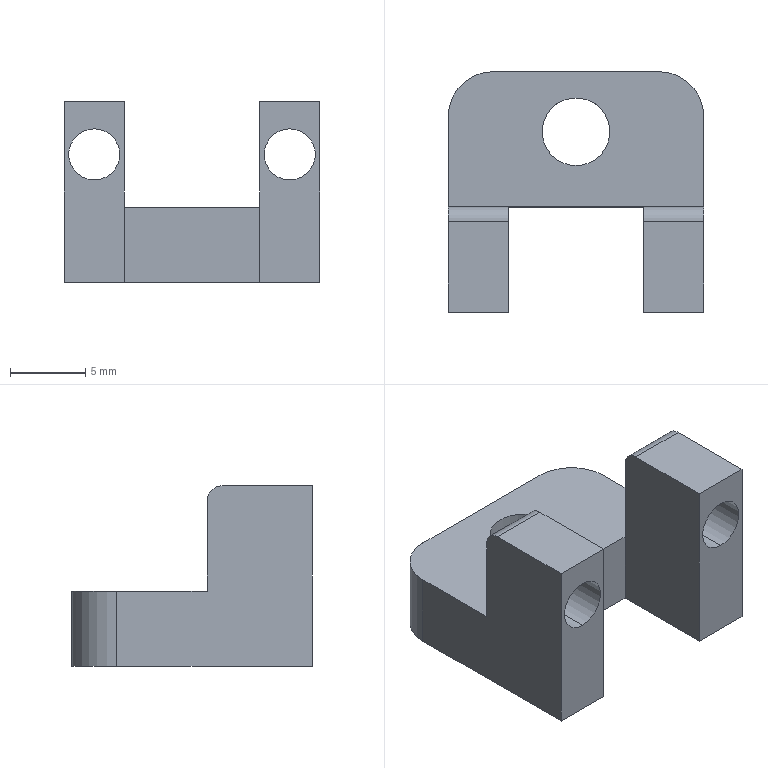Component | SolidWorks | MGL-PACK-01-00WeldedPlate1Assembly-1_MGL-PACK-01-03FixingBlock-1 | 1 solid | 24 faces | box 17 x 16 x 12 mm | volume 1209 mm3 | plane 14 | cylinder 10 | commonest cylinder face diameters 3.4 x4 4.5 x2 6 x2 2 x2
STEP:
#1=COLOUR_RGB('',0.7922,0.8196,0.9333);
#2=FILL_AREA_STYLE_COLOUR('',#1);
#3=FILL_AREA_STYLE('',(#2));
#4=SURFACE_STYLE_FILL_AREA(#3);
#5=SURFACE_SIDE_STYLE('',(#4));
#6=SURFACE_STYLE_USAGE(.BOTH.,#5);
#7=PRESENTATION_STYLE_ASSIGNMENT((#6));
#8=CARTESIAN_POINT('',(-3.585,1.831,0.2677));
#9=VERTEX_POINT('',#8);
#10=CARTESIAN_POINT('',(-3.585,1.831,0.4016));
#11=VERTEX_POINT('',#10);
#12=CARTESIAN_POINT('',(-3.585,1.831,0.3346));
#13=DIRECTION('',(-0.,1.,0.));
#14=DIRECTION('',(-1.,0.,0.));
#15=AXIS2_PLACEMENT_3D('',#12,#13,#14);
#16=CIRCLE('',#15,0.06693);
#17=EDGE_CURVE('',#9,#11,#16,.T.);
#18=ORIENTED_EDGE('',*,*,#17,.F.);
#19=CARTESIAN_POINT('',(-3.585,2.106,0.2677));
#20=VERTEX_POINT('',#19);
#21=CARTESIAN_POINT('',(-3.585,2.106,0.2677));
#22=DIRECTION('',(0.,1.,0.));
#23=VECTOR('',#22,39.37);
#24=LINE('',#21,#23);
#25=EDGE_CURVE('',#9,#20,#24,.T.);
#26=ORIENTED_EDGE('',*,*,#25,.T.);
#27=CARTESIAN_POINT('',(-3.585,2.106,0.4016));
#28=VERTEX_POINT('',#27);
#29=CARTESIAN_POINT('',(-3.585,2.106,0.3346));
#30=DIRECTION('',(0.,1.,0.));
#31=DIRECTION('',(0.,0.,1.));
#32=AXIS2_PLACEMENT_3D('',#29,#30,#31);
#33=CIRCLE('',#32,0.06693);
#34=EDGE_CURVE('',#20,#28,#33,.T.);
#35=ORIENTED_EDGE('',*,*,#34,.T.);
#36=CARTESIAN_POINT('',(-3.585,2.106,0.4016));
#37=DIRECTION('',(0.,1.,0.));
#38=VECTOR('',#37,39.37);
#39=LINE('',#36,#38);
#40=EDGE_CURVE('',#11,#28,#39,.T.);
#41=ORIENTED_EDGE('',*,*,#40,.F.);
#42=EDGE_LOOP('',(#18,#26,#35,#41));
#43=FACE_OUTER_BOUND('',#42,.T.);
#44=CARTESIAN_POINT('',(-3.585,2.106,0.3346));
#45=DIRECTION('',(0.,1.,0.));
#46=DIRECTION('',(0.,0.,1.));
#47=AXIS2_PLACEMENT_3D('',#44,#45,#46);
#48=CYLINDRICAL_SURFACE('',#47,0.06693);
#49=ADVANCED_FACE('',(#43),#48,.F.);
#50=CARTESIAN_POINT('',(-3.073,1.831,0.2677));
#51=VERTEX_POINT('',#50);
#52=CARTESIAN_POINT('',(-3.073,1.831,0.4016));
#53=VERTEX_POINT('',#52);
#54=CARTESIAN_POINT('',(-3.073,1.831,0.3346));
#55=DIRECTION('',(0.,1.,0.));
#56=DIRECTION('',(-1.,0.,0.));
#57=AXIS2_PLACEMENT_3D('',#54,#55,#56);
#58=CIRCLE('',#57,0.06693);
#59=EDGE_CURVE('',#51,#53,#58,.T.);
#60=ORIENTED_EDGE('',*,*,#59,.F.);
#61=CARTESIAN_POINT('',(-3.073,2.106,0.2677));
#62=VERTEX_POINT('',#61);
#63=CARTESIAN_POINT('',(-3.073,2.106,0.2677));
#64=DIRECTION('',(0.,1.,0.));
#65=VECTOR('',#64,39.37);
#66=LINE('',#63,#65);
#67=EDGE_CURVE('',#51,#62,#66,.T.);
#68=ORIENTED_EDGE('',*,*,#67,.T.);
#69=CARTESIAN_POINT('',(-3.073,2.106,0.4016));
#70=VERTEX_POINT('',#69);
#71=CARTESIAN_POINT('',(-3.073,2.106,0.3346));
#72=DIRECTION('',(0.,1.,0.));
#73=DIRECTION('',(0.,0.,1.));
#74=AXIS2_PLACEMENT_3D('',#71,#72,#73);
#75=CIRCLE('',#74,0.06693);
#76=EDGE_CURVE('',#62,#70,#75,.T.);
#77=ORIENTED_EDGE('',*,*,#76,.T.);
#78=CARTESIAN_POINT('',(-3.073,2.106,0.4016));
#79=DIRECTION('',(0.,1.,0.));
#80=VECTOR('',#79,39.37);
#81=LINE('',#78,#80);
#82=EDGE_CURVE('',#53,#70,#81,.T.);
#83=ORIENTED_EDGE('',*,*,#82,.F.);
#84=EDGE_LOOP('',(#60,#68,#77,#83));
#85=FACE_OUTER_BOUND('',#84,.T.);
#86=CARTESIAN_POINT('',(-3.073,2.106,0.3346));
#87=DIRECTION('',(0.,1.,0.));
#88=DIRECTION('',(0.,0.,1.));
#89=AXIS2_PLACEMENT_3D('',#86,#87,#88);
#90=CYLINDRICAL_SURFACE('',#89,0.06693);
#91=ADVANCED_FACE('',(#85),#90,.F.);
#92=CARTESIAN_POINT('',(-3.417,2.303,0.));
#93=VERTEX_POINT('',#92);
#94=CARTESIAN_POINT('',(-3.24,2.303,0.));
#95=VERTEX_POINT('',#94);
#96=CARTESIAN_POINT('',(-3.329,2.303,0.));
#97=DIRECTION('',(0.,0.,1.));
#98=DIRECTION('',(1.,0.,0.));
#99=AXIS2_PLACEMENT_3D('',#96,#97,#98);
#100=CIRCLE('',#99,0.08858);
#101=EDGE_CURVE('',#93,#95,#100,.T.);
#102=ORIENTED_EDGE('',*,*,#101,.F.);
#103=CARTESIAN_POINT('',(-3.417,2.303,0.1969));
#104=VERTEX_POINT('',#103);
#105=CARTESIAN_POINT('',(-3.417,2.303,0.1969));
#106=DIRECTION('',(0.,0.,1.));
#107=VECTOR('',#106,39.37);
#108=LINE('',#105,#107);
#109=EDGE_CURVE('',#93,#104,#108,.T.);
#110=ORIENTED_EDGE('',*,*,#109,.T.);
#111=CARTESIAN_POINT('',(-3.24,2.303,0.1969));
#112=VERTEX_POINT('',#111);
#113=CARTESIAN_POINT('',(-3.329,2.303,0.1969));
#114=DIRECTION('',(0.,0.,1.));
#115=DIRECTION('',(1.,0.,0.));
#116=AXIS2_PLACEMENT_3D('',#113,#114,#115);
#117=CIRCLE('',#116,0.08858);
#118=EDGE_CURVE('',#104,#112,#117,.T.);
#119=ORIENTED_EDGE('',*,*,#118,.T.);
#120=CARTESIAN_POINT('',(-3.24,2.303,0.1969));
#121=DIRECTION('',(0.,0.,1.));
#122=VECTOR('',#121,39.37);
#123=LINE('',#120,#122);
#124=EDGE_CURVE('',#95,#112,#123,.T.);
#125=ORIENTED_EDGE('',*,*,#124,.F.);
#126=EDGE_LOOP('',(#102,#110,#119,#125));
#127=FACE_OUTER_BOUND('',#126,.T.);
#128=CARTESIAN_POINT('',(-3.329,2.303,0.1969));
#129=DIRECTION('',(0.,0.,1.));
#130=DIRECTION('',(1.,0.,0.));
#131=AXIS2_PLACEMENT_3D('',#128,#129,#130);
#132=CYLINDRICAL_SURFACE('',#131,0.08858);
#133=ADVANCED_FACE('',(#127),#132,.F.);
#134=CARTESIAN_POINT('',(-3.506,1.831,0.4724));
#135=VERTEX_POINT('',#134);
#136=CARTESIAN_POINT('',(-3.506,2.067,0.4724));
#137=VERTEX_POINT('',#136);
#138=CARTESIAN_POINT('',(-3.506,1.831,0.4724));
#139=DIRECTION('',(0.,1.,0.));
#140=VECTOR('',#139,39.37);
#141=LINE('',#138,#140);
#142=EDGE_CURVE('',#135,#137,#141,.T.);
#143=ORIENTED_EDGE('',*,*,#142,.T.);
#144=CARTESIAN_POINT('',(-3.663,2.067,0.4724));
#145=VERTEX_POINT('',#144);
#146=CARTESIAN_POINT('',(-3.663,2.067,0.4724));
#147=DIRECTION('',(-1.,0.,0.));
#148=VECTOR('',#147,39.37);
#149=LINE('',#146,#148);
#150=EDGE_CURVE('',#137,#145,#149,.T.);
#151=ORIENTED_EDGE('',*,*,#150,.T.);
#152=CARTESIAN_POINT('',(-3.663,1.831,0.4724));
#153=VERTEX_POINT('',#152);
#154=CARTESIAN_POINT('',(-3.663,2.461,0.4724));
#155=DIRECTION('',(-0.,-1.,0.));
#156=VECTOR('',#155,39.37);
#157=LINE('',#154,#156);
#158=EDGE_CURVE('',#145,#153,#157,.T.);
#159=ORIENTED_EDGE('',*,*,#158,.T.);
#160=CARTESIAN_POINT('',(-3.663,1.831,0.4724));
#161=DIRECTION('',(1.,0.,0.));
#162=VECTOR('',#161,39.37);
#163=LINE('',#160,#162);
#164=EDGE_CURVE('',#153,#135,#163,.T.);
#165=ORIENTED_EDGE('',*,*,#164,.T.);
#166=EDGE_LOOP('',(#143,#151,#159,#165));
#167=FACE_OUTER_BOUND('',#166,.T.);
#168=CARTESIAN_POINT('',(-3.329,2.146,0.4724));
#169=DIRECTION('',(0.,0.,1.));
#170=DIRECTION('',(1.,0.,0.));
#171=AXIS2_PLACEMENT_3D('',#168,#169,#170);
#172=PLANE('',#171);
#173=ADVANCED_FACE('',(#167),#172,.T.);
#174=ORIENTED_EDGE('',*,*,#158,.F.);
#175=CARTESIAN_POINT('',(-3.663,2.106,0.4331));
#176=VERTEX_POINT('',#175);
#177=CARTESIAN_POINT('',(-3.663,2.067,0.4331));
#178=DIRECTION('',(-1.,0.,0.));
#179=DIRECTION('',(0.,1.,0.));
#180=AXIS2_PLACEMENT_3D('',#177,#178,#179);
#181=CIRCLE('',#180,0.03937);
#182=EDGE_CURVE('',#145,#176,#181,.T.);
#183=ORIENTED_EDGE('',*,*,#182,.T.);
#184=CARTESIAN_POINT('',(-3.663,2.106,0.1969));
#185=VERTEX_POINT('',#184);
#186=CARTESIAN_POINT('',(-3.663,2.106,0.1969));
#187=DIRECTION('',(0.,0.,1.));
#188=VECTOR('',#187,39.37);
#189=LINE('',#186,#188);
#190=EDGE_CURVE('',#185,#176,#189,.T.);
#191=ORIENTED_EDGE('',*,*,#190,.F.);
#192=CARTESIAN_POINT('',(-3.663,2.343,0.1969));
#193=VERTEX_POINT('',#192);
#194=CARTESIAN_POINT('',(-3.663,2.106,0.1969));
#195=DIRECTION('',(0.,-1.,0.));
#196=VECTOR('',#195,39.37);
#197=LINE('',#194,#196);
#198=EDGE_CURVE('',#193,#185,#197,.T.);
#199=ORIENTED_EDGE('',*,*,#198,.F.);
#200=CARTESIAN_POINT('',(-3.663,2.343,0.));
#201=VERTEX_POINT('',#200);
#202=CARTESIAN_POINT('',(-3.663,2.343,0.4724));
#203=DIRECTION('',(0.,0.,-1.));
#204=VECTOR('',#203,39.37);
#205=LINE('',#202,#204);
#206=EDGE_CURVE('',#193,#201,#205,.T.);
#207=ORIENTED_EDGE('',*,*,#206,.T.);
#208=CARTESIAN_POINT('',(-3.663,1.831,0.));
#209=VERTEX_POINT('',#208);
#210=CARTESIAN_POINT('',(-3.663,2.461,0.));
#211=DIRECTION('',(-0.,-1.,0.));
#212=VECTOR('',#211,39.37);
#213=LINE('',#210,#212);
#214=EDGE_CURVE('',#201,#209,#213,.T.);
#215=ORIENTED_EDGE('',*,*,#214,.T.);
#216=CARTESIAN_POINT('',(-3.663,1.831,0.4724));
#217=DIRECTION('',(0.,0.,-1.));
#218=VECTOR('',#217,39.37);
#219=LINE('',#216,#218);
#220=EDGE_CURVE('',#153,#209,#219,.T.);
#221=ORIENTED_EDGE('',*,*,#220,.F.);
#222=EDGE_LOOP('',(#174,#183,#191,#199,#207,#215,#221));
#223=FACE_OUTER_BOUND('',#222,.T.);
#224=CARTESIAN_POINT('',(-3.663,2.461,0.4724));
#225=DIRECTION('',(1.,-0.,0.));
#226=DIRECTION('',(0.,1.,0.));
#227=AXIS2_PLACEMENT_3D('',#224,#225,#226);
#228=PLANE('',#227);
#229=ADVANCED_FACE('',(#223),#228,.F.);
#230=CARTESIAN_POINT('',(-3.585,1.831,0.3346));
#231=DIRECTION('',(-0.,1.,0.));
#232=DIRECTION('',(-1.,0.,0.));
#233=AXIS2_PLACEMENT_3D('',#230,#231,#232);
#234=CIRCLE('',#233,0.06693);
#235=EDGE_CURVE('',#11,#9,#234,.T.);
#236=ORIENTED_EDGE('',*,*,#235,.T.);
#237=ORIENTED_EDGE('',*,*,#17,.T.);
#238=EDGE_LOOP('',(#236,#237));
#239=FACE_BOUND('',#238,.T.);
#240=CARTESIAN_POINT('',(-3.506,1.831,0.));
#241=VERTEX_POINT('',#240);
#242=CARTESIAN_POINT('',(-3.663,1.831,0.));
#243=DIRECTION('',(1.,0.,0.));
#244=VECTOR('',#243,39.37);
#245=LINE('',#242,#244);
#246=EDGE_CURVE('',#209,#241,#245,.T.);
#247=ORIENTED_EDGE('',*,*,#246,.T.);
#248=CARTESIAN_POINT('',(-3.506,1.831,0.4724));
#249=DIRECTION('',(0.,0.,-1.));
#250=VECTOR('',#249,39.37);
#251=LINE('',#248,#250);
#252=EDGE_CURVE('',#135,#241,#251,.T.);
#253=ORIENTED_EDGE('',*,*,#252,.F.);
#254=ORIENTED_EDGE('',*,*,#164,.F.);
#255=ORIENTED_EDGE('',*,*,#220,.T.);
#256=EDGE_LOOP('',(#247,#253,#254,#255));
#257=FACE_OUTER_BOUND('',#256,.T.);
#258=CARTESIAN_POINT('',(-3.663,1.831,0.4724));
#259=DIRECTION('',(-0.,1.,0.));
#260=DIRECTION('',(-1.,-0.,0.));
#261=AXIS2_PLACEMENT_3D('',#258,#259,#260);
#262=PLANE('',#261);
#263=ADVANCED_FACE('',(#239,#257),#262,.F.);
#264=CARTESIAN_POINT('',(-3.506,2.106,0.4331));
#265=VERTEX_POINT('',#264);
#266=CARTESIAN_POINT('',(-3.506,2.106,0.1969));
#267=VERTEX_POINT('',#266);
#268=CARTESIAN_POINT('',(-3.506,2.106,0.4724));
#269=DIRECTION('',(0.,0.,-1.));
#270=VECTOR('',#269,39.37);
#271=LINE('',#268,#270);
#272=EDGE_CURVE('',#265,#267,#271,.T.);
#273=ORIENTED_EDGE('',*,*,#272,.F.);
#274=CARTESIAN_POINT('',(-3.506,2.067,0.4331));
#275=DIRECTION('',(1.,0.,0.));
#276=DIRECTION('',(0.,0.,1.));
#277=AXIS2_PLACEMENT_3D('',#274,#275,#276);
#278=CIRCLE('',#277,0.03937);
#279=EDGE_CURVE('',#265,#137,#278,.T.);
#280=ORIENTED_EDGE('',*,*,#279,.T.);
#281=ORIENTED_EDGE('',*,*,#142,.F.);
#282=ORIENTED_EDGE('',*,*,#252,.T.);
#283=CARTESIAN_POINT('',(-3.506,2.106,0.));
#284=VERTEX_POINT('',#283);
#285=CARTESIAN_POINT('',(-3.506,1.831,0.));
#286=DIRECTION('',(0.,1.,0.));
#287=VECTOR('',#286,39.37);
#288=LINE('',#285,#287);
#289=EDGE_CURVE('',#241,#284,#288,.T.);
#290=ORIENTED_EDGE('',*,*,#289,.T.);
#291=CARTESIAN_POINT('',(-3.506,2.106,0.4724));
#292=DIRECTION('',(0.,0.,-1.));
#293=VECTOR('',#292,39.37);
#294=LINE('',#291,#293);
#295=EDGE_CURVE('',#267,#284,#294,.T.);
#296=ORIENTED_EDGE('',*,*,#295,.F.);
#297=EDGE_LOOP('',(#273,#280,#281,#282,#290,#296));
#298=FACE_OUTER_BOUND('',#297,.T.);
#299=CARTESIAN_POINT('',(-3.506,1.831,0.4724));
#300=DIRECTION('',(-1.,0.,0.));
#301=DIRECTION('',(0.,0.,1.));
#302=AXIS2_PLACEMENT_3D('',#299,#300,#301);
#303=PLANE('',#302);
#304=ADVANCED_FACE('',(#298),#303,.F.);
#305=CARTESIAN_POINT('',(-3.152,2.106,0.1969));
#306=VERTEX_POINT('',#305);
#307=CARTESIAN_POINT('',(-3.152,2.106,0.));
#308=VERTEX_POINT('',#307);
#309=CARTESIAN_POINT('',(-3.152,2.106,0.4724));
#310=DIRECTION('',(0.,0.,-1.));
#311=VECTOR('',#310,39.37);
#312=LINE('',#309,#311);
#313=EDGE_CURVE('',#306,#308,#312,.T.);
#314=ORIENTED_EDGE('',*,*,#313,.F.);
#315=CARTESIAN_POINT('',(-3.506,2.106,0.1969));
#316=DIRECTION('',(1.,0.,0.));
#317=VECTOR('',#316,39.37);
#318=LINE('',#315,#317);
#319=EDGE_CURVE('',#267,#306,#318,.T.);
#320=ORIENTED_EDGE('',*,*,#319,.F.);
#321=ORIENTED_EDGE('',*,*,#295,.T.);
#322=CARTESIAN_POINT('',(-3.506,2.106,0.));
#323=DIRECTION('',(1.,0.,0.));
#324=VECTOR('',#323,39.37);
#325=LINE('',#322,#324);
#326=EDGE_CURVE('',#284,#308,#325,.T.);
#327=ORIENTED_EDGE('',*,*,#326,.T.);
#328=EDGE_LOOP('',(#314,#320,#321,#327));
#329=FACE_OUTER_BOUND('',#328,.T.);
#330=CARTESIAN_POINT('',(-3.506,2.106,0.4724));
#331=DIRECTION('',(0.,1.,0.));
#332=DIRECTION('',(0.,0.,1.));
#333=AXIS2_PLACEMENT_3D('',#330,#331,#332);
#334=PLANE('',#333);
#335=ADVANCED_FACE('',(#329),#334,.F.);
#336=CARTESIAN_POINT('',(-3.152,2.067,0.4724));
#337=VERTEX_POINT('',#336);
#338=CARTESIAN_POINT('',(-3.152,1.831,0.4724));
#339=VERTEX_POINT('',#338);
#340=CARTESIAN_POINT('',(-3.152,2.106,0.4724));
#341=DIRECTION('',(0.,-1.,0.));
#342=VECTOR('',#341,39.37);
#343=LINE('',#340,#342);
#344=EDGE_CURVE('',#337,#339,#343,.T.);
#345=ORIENTED_EDGE('',*,*,#344,.F.);
#346=CARTESIAN_POINT('',(-3.152,2.106,0.4331));
#347=VERTEX_POINT('',#346);
#348=CARTESIAN_POINT('',(-3.152,2.067,0.4331));
#349=DIRECTION('',(-1.,0.,0.));
#350=DIRECTION('',(0.,0.,-1.));
#351=AXIS2_PLACEMENT_3D('',#348,#349,#350);
#352=CIRCLE('',#351,0.03937);
#353=EDGE_CURVE('',#337,#347,#352,.T.);
#354=ORIENTED_EDGE('',*,*,#353,.T.);
#355=CARTESIAN_POINT('',(-3.152,2.106,0.4724));
#356=DIRECTION('',(0.,0.,-1.));
#357=VECTOR('',#356,39.37);
#358=LINE('',#355,#357);
#359=EDGE_CURVE('',#347,#306,#358,.T.);
#360=ORIENTED_EDGE('',*,*,#359,.T.);
#361=ORIENTED_EDGE('',*,*,#313,.T.);
#362=CARTESIAN_POINT('',(-3.152,1.831,0.));
#363=VERTEX_POINT('',#362);
#364=CARTESIAN_POINT('',(-3.152,2.106,0.));
#365=DIRECTION('',(0.,-1.,0.));
#366=VECTOR('',#365,39.37);
#367=LINE('',#364,#366);
#368=EDGE_CURVE('',#308,#363,#367,.T.);
#369=ORIENTED_EDGE('',*,*,#368,.T.);
#370=CARTESIAN_POINT('',(-3.152,1.831,0.4724));
#371=DIRECTION('',(0.,0.,-1.));
#372=VECTOR('',#371,39.37);
#373=LINE('',#370,#372);
#374=EDGE_CURVE('',#339,#363,#373,.T.);
#375=ORIENTED_EDGE('',*,*,#374,.F.);
#376=EDGE_LOOP('',(#345,#354,#360,#361,#369,#375));
#377=FACE_OUTER_BOUND('',#376,.T.);
#378=CARTESIAN_POINT('',(-3.152,2.106,0.4724));
#379=DIRECTION('',(1.,0.,0.));
#380=DIRECTION('',(0.,0.,-1.));
#381=AXIS2_PLACEMENT_3D('',#378,#379,#380);
#382=PLANE('',#381);
#383=ADVANCED_FACE('',(#377),#382,.F.);
#384=CARTESIAN_POINT('',(-3.073,1.831,0.3346));
#385=DIRECTION('',(0.,1.,0.));
#386=DIRECTION('',(-1.,0.,0.));
#387=AXIS2_PLACEMENT_3D('',#384,#385,#386);
#388=CIRCLE('',#387,0.06693);
#389=EDGE_CURVE('',#53,#51,#388,.T.);
#390=ORIENTED_EDGE('',*,*,#389,.T.);
#391=ORIENTED_EDGE('',*,*,#59,.T.);
#392=EDGE_LOOP('',(#390,#391));
#393=FACE_BOUND('',#392,.T.);
#394=CARTESIAN_POINT('',(-2.994,1.831,0.));
#395=VERTEX_POINT('',#394);
#396=CARTESIAN_POINT('',(-3.152,1.831,0.));
#397=DIRECTION('',(1.,-0.,0.));
#398=VECTOR('',#397,39.37);
#399=LINE('',#396,#398);
#400=EDGE_CURVE('',#363,#395,#399,.T.);
#401=ORIENTED_EDGE('',*,*,#400,.T.);
#402=CARTESIAN_POINT('',(-2.994,1.831,0.4724));
#403=VERTEX_POINT('',#402);
#404=CARTESIAN_POINT('',(-2.994,1.831,0.4724));
#405=DIRECTION('',(0.,0.,-1.));
#406=VECTOR('',#405,39.37);
#407=LINE('',#404,#406);
#408=EDGE_CURVE('',#403,#395,#407,.T.);
#409=ORIENTED_EDGE('',*,*,#408,.F.);
#410=CARTESIAN_POINT('',(-3.152,1.831,0.4724));
#411=DIRECTION('',(1.,-0.,0.));
#412=VECTOR('',#411,39.37);
#413=LINE('',#410,#412);
#414=EDGE_CURVE('',#339,#403,#413,.T.);
#415=ORIENTED_EDGE('',*,*,#414,.F.);
#416=ORIENTED_EDGE('',*,*,#374,.T.);
#417=EDGE_LOOP('',(#401,#409,#415,#416));
#418=FACE_OUTER_BOUND('',#417,.T.);
#419=CARTESIAN_POINT('',(-3.152,1.831,0.4724));
#420=DIRECTION('',(0.,1.,0.));
#421=DIRECTION('',(-1.,0.,0.));
#422=AXIS2_PLACEMENT_3D('',#419,#420,#421);
#423=PLANE('',#422);
#424=ADVANCED_FACE('',(#393,#418),#423,.F.);
#425=CARTESIAN_POINT('',(-2.994,2.106,0.1969));
#426=VERTEX_POINT('',#425);
#427=CARTESIAN_POINT('',(-2.994,2.106,0.4331));
#428=VERTEX_POINT('',#427);
#429=CARTESIAN_POINT('',(-2.994,2.106,0.1969));
#430=DIRECTION('',(0.,0.,1.));
#431=VECTOR('',#430,39.37);
#432=LINE('',#429,#431);
#433=EDGE_CURVE('',#426,#428,#432,.T.);
#434=ORIENTED_EDGE('',*,*,#433,.T.);
#435=CARTESIAN_POINT('',(-2.994,2.067,0.4724));
#436=VERTEX_POINT('',#435);
#437=CARTESIAN_POINT('',(-2.994,2.067,0.4331));
#438=DIRECTION('',(1.,-0.,0.));
#439=DIRECTION('',(0.,-1.,0.));
#440=AXIS2_PLACEMENT_3D('',#437,#438,#439);
#441=CIRCLE('',#440,0.03937);
#442=EDGE_CURVE('',#428,#436,#441,.T.);
#443=ORIENTED_EDGE('',*,*,#442,.T.);
#444=CARTESIAN_POINT('',(-2.994,2.461,0.4724));
#445=DIRECTION('',(0.,1.,0.));
#446=VECTOR('',#445,39.37);
#447=LINE('',#444,#446);
#448=EDGE_CURVE('',#403,#436,#447,.T.);
#449=ORIENTED_EDGE('',*,*,#448,.F.);
#450=ORIENTED_EDGE('',*,*,#408,.T.);
#451=CARTESIAN_POINT('',(-2.994,2.343,0.));
#452=VERTEX_POINT('',#451);
#453=CARTESIAN_POINT('',(-2.994,2.461,0.));
#454=DIRECTION('',(0.,1.,0.));
#455=VECTOR('',#454,39.37);
#456=LINE('',#453,#455);
#457=EDGE_CURVE('',#395,#452,#456,.T.);
#458=ORIENTED_EDGE('',*,*,#457,.T.);
#459=CARTESIAN_POINT('',(-2.994,2.343,0.1969));
#460=VERTEX_POINT('',#459);
#461=CARTESIAN_POINT('',(-2.994,2.343,0.4724));
#462=DIRECTION('',(0.,0.,1.));
#463=VECTOR('',#462,39.37);
#464=LINE('',#461,#463);
#465=EDGE_CURVE('',#452,#460,#464,.T.);
#466=ORIENTED_EDGE('',*,*,#465,.T.);
#467=CARTESIAN_POINT('',(-2.994,2.343,0.1969));
#468=DIRECTION('',(0.,1.,0.));
#469=VECTOR('',#468,39.37);
#470=LINE('',#467,#469);
#471=EDGE_CURVE('',#426,#460,#470,.T.);
#472=ORIENTED_EDGE('',*,*,#471,.F.);
#473=EDGE_LOOP('',(#434,#443,#449,#450,#458,#466,#472));
#474=FACE_OUTER_BOUND('',#473,.T.);
#475=CARTESIAN_POINT('',(-2.994,2.461,0.4724));
#476=DIRECTION('',(-1.,0.,0.));
#477=DIRECTION('',(-0.,-1.,0.));
#478=AXIS2_PLACEMENT_3D('',#475,#476,#477);
#479=PLANE('',#478);
#480=ADVANCED_FACE('',(#474),#479,.F.);
#481=CARTESIAN_POINT('',(-3.545,2.461,0.));
#482=VERTEX_POINT('',#481);
#483=CARTESIAN_POINT('',(-3.545,2.461,0.1969));
#484=VERTEX_POINT('',#483);
#485=CARTESIAN_POINT('',(-3.545,2.461,0.4724));
#486=DIRECTION('',(0.,0.,1.));
#487=VECTOR('',#486,39.37);
#488=LINE('',#485,#487);
#489=EDGE_CURVE('',#482,#484,#488,.T.);
#490=ORIENTED_EDGE('',*,*,#489,.T.);
#491=CARTESIAN_POINT('',(-3.112,2.461,0.1969));
#492=VERTEX_POINT('',#491);
#493=CARTESIAN_POINT('',(-3.545,2.461,0.1969));
#494=DIRECTION('',(-1.,0.,0.));
#495=VECTOR('',#494,39.37);
#496=LINE('',#493,#495);
#497=EDGE_CURVE('',#492,#484,#496,.T.);
#498=ORIENTED_EDGE('',*,*,#497,.F.);
#499=CARTESIAN_POINT('',(-3.112,2.461,0.));
#500=VERTEX_POINT('',#499);
#501=CARTESIAN_POINT('',(-3.112,2.461,0.4724));
#502=DIRECTION('',(0.,0.,-1.));
#503=VECTOR('',#502,39.37);
#504=LINE('',#501,#503);
#505=EDGE_CURVE('',#492,#500,#504,.T.);
#506=ORIENTED_EDGE('',*,*,#505,.T.);
#507=CARTESIAN_POINT('',(-3.663,2.461,0.));
#508=DIRECTION('',(-1.,0.,0.));
#509=VECTOR('',#508,39.37);
#510=LINE('',#507,#509);
#511=EDGE_CURVE('',#500,#482,#510,.T.);
#512=ORIENTED_EDGE('',*,*,#511,.T.);
#513=EDGE_LOOP('',(#490,#498,#506,#512));
#514=FACE_OUTER_BOUND('',#513,.T.);
#515=CARTESIAN_POINT('',(-3.663,2.461,0.4724));
#516=DIRECTION('',(0.,-1.,0.));
#517=DIRECTION('',(0.,0.,-1.));
#518=AXIS2_PLACEMENT_3D('',#515,#516,#517);
#519=PLANE('',#518);
#520=ADVANCED_FACE('',(#514),#519,.F.);
#521=ORIENTED_EDGE('',*,*,#448,.T.);
#522=CARTESIAN_POINT('',(-3.152,2.067,0.4724));
#523=DIRECTION('',(-1.,0.,0.));
#524=VECTOR('',#523,39.37);
#525=LINE('',#522,#524);
#526=EDGE_CURVE('',#436,#337,#525,.T.);
#527=ORIENTED_EDGE('',*,*,#526,.T.);
#528=ORIENTED_EDGE('',*,*,#344,.T.);
#529=ORIENTED_EDGE('',*,*,#414,.T.);
#530=EDGE_LOOP('',(#521,#527,#528,#529));
#531=FACE_OUTER_BOUND('',#530,.T.);
#532=CARTESIAN_POINT('',(-3.329,2.146,0.4724));
#533=DIRECTION('',(0.,0.,1.));
#534=DIRECTION('',(1.,0.,0.));
#535=AXIS2_PLACEMENT_3D('',#532,#533,#534);
#536=PLANE('',#535);
#537=ADVANCED_FACE('',(#531),#536,.T.);
#538=CARTESIAN_POINT('',(-3.329,2.303,0.));
#539=DIRECTION('',(0.,0.,1.));
#540=DIRECTION('',(1.,0.,0.));
#541=AXIS2_PLACEMENT_3D('',#538,#539,#540);
#542=CIRCLE('',#541,0.08858);
#543=EDGE_CURVE('',#95,#93,#542,.T.);
#544=ORIENTED_EDGE('',*,*,#543,.T.);
#545=ORIENTED_EDGE('',*,*,#101,.T.);
#546=EDGE_LOOP('',(#544,#545));
#547=FACE_BOUND('',#546,.T.);
#548=ORIENTED_EDGE('',*,*,#511,.F.);
#549=CARTESIAN_POINT('',(-3.112,2.343,0.));
#550=DIRECTION('',(0.,0.,-1.));
#551=DIRECTION('',(1.,0.,0.));
#552=AXIS2_PLACEMENT_3D('',#549,#550,#551);
#553=CIRCLE('',#552,0.1181);
#554=EDGE_CURVE('',#500,#452,#553,.T.);
#555=ORIENTED_EDGE('',*,*,#554,.T.);
#556=ORIENTED_EDGE('',*,*,#457,.F.);
#557=ORIENTED_EDGE('',*,*,#400,.F.);
#558=ORIENTED_EDGE('',*,*,#368,.F.);
#559=ORIENTED_EDGE('',*,*,#326,.F.);
#560=ORIENTED_EDGE('',*,*,#289,.F.);
#561=ORIENTED_EDGE('',*,*,#246,.F.);
#562=ORIENTED_EDGE('',*,*,#214,.F.);
#563=CARTESIAN_POINT('',(-3.545,2.343,0.));
#564=DIRECTION('',(0.,0.,-1.));
#565=DIRECTION('',(1.,0.,0.));
#566=AXIS2_PLACEMENT_3D('',#563,#564,#565);
#567=CIRCLE('',#566,0.1181);
#568=EDGE_CURVE('',#201,#482,#567,.T.);
#569=ORIENTED_EDGE('',*,*,#568,.T.);
#570=EDGE_LOOP('',(#548,#555,#556,#557,#558,#559,#560,#561,#562,#569));
#571=FACE_OUTER_BOUND('',#570,.T.);
#572=CARTESIAN_POINT('',(-3.329,2.146,0.));
#573=DIRECTION('',(0.,0.,1.));
#574=DIRECTION('',(1.,0.,0.));
#575=AXIS2_PLACEMENT_3D('',#572,#573,#574);
#576=PLANE('',#575);
#577=ADVANCED_FACE('',(#547,#571),#576,.F.);
#578=CARTESIAN_POINT('',(-3.112,2.343,0.1969));
#579=DIRECTION('',(0.,0.,1.));
#580=DIRECTION('',(-1.,0.,0.));
#581=AXIS2_PLACEMENT_3D('',#578,#579,#580);
#582=CIRCLE('',#581,0.1181);
#583=EDGE_CURVE('',#460,#492,#582,.T.);
#584=ORIENTED_EDGE('',*,*,#583,.F.);
#585=ORIENTED_EDGE('',*,*,#465,.F.);
#586=ORIENTED_EDGE('',*,*,#554,.F.);
#587=ORIENTED_EDGE('',*,*,#505,.F.);
#588=EDGE_LOOP('',(#584,#585,#586,#587));
#589=FACE_OUTER_BOUND('',#588,.T.);
#590=CARTESIAN_POINT('',(-3.112,2.343,0.4724));
#591=DIRECTION('',(0.,0.,-1.));
#592=DIRECTION('',(-1.,0.,0.));
#593=AXIS2_PLACEMENT_3D('',#590,#591,#592);
#594=CYLINDRICAL_SURFACE('',#593,0.1181);
#595=ADVANCED_FACE('',(#589),#594,.T.);
#596=CARTESIAN_POINT('',(-3.545,2.343,0.1969));
#597=DIRECTION('',(0.,0.,1.));
#598=DIRECTION('',(-1.,0.,0.));
#599=AXIS2_PLACEMENT_3D('',#596,#597,#598);
#600=CIRCLE('',#599,0.1181);
#601=EDGE_CURVE('',#484,#193,#600,.T.);
#602=ORIENTED_EDGE('',*,*,#601,.F.);
#603=ORIENTED_EDGE('',*,*,#489,.F.);
#604=ORIENTED_EDGE('',*,*,#568,.F.);
#605=ORIENTED_EDGE('',*,*,#206,.F.);
#606=EDGE_LOOP('',(#602,#603,#604,#605));
#607=FACE_OUTER_BOUND('',#606,.T.);
#608=CARTESIAN_POINT('',(-3.545,2.343,0.4724));
#609=DIRECTION('',(0.,0.,-1.));
#610=DIRECTION('',(-1.,0.,0.));
#611=AXIS2_PLACEMENT_3D('',#608,#609,#610);
#612=CYLINDRICAL_SURFACE('',#611,0.1181);
#613=ADVANCED_FACE('',(#607),#612,.T.);
#614=CARTESIAN_POINT('',(-3.585,2.106,0.3346));
#615=DIRECTION('',(0.,1.,0.));
#616=DIRECTION('',(0.,0.,1.));
#617=AXIS2_PLACEMENT_3D('',#614,#615,#616);
#618=CIRCLE('',#617,0.06693);
#619=EDGE_CURVE('',#28,#20,#618,.T.);
#620=ORIENTED_EDGE('',*,*,#619,.F.);
#621=ORIENTED_EDGE('',*,*,#34,.F.);
#622=EDGE_LOOP('',(#620,#621));
#623=FACE_BOUND('',#622,.T.);
#624=ORIENTED_EDGE('',*,*,#190,.T.);
#625=CARTESIAN_POINT('',(-3.506,2.106,0.4331));
#626=DIRECTION('',(1.,0.,0.));
#627=VECTOR('',#626,39.37);
#628=LINE('',#625,#627);
#629=EDGE_CURVE('',#176,#265,#628,.T.);
#630=ORIENTED_EDGE('',*,*,#629,.T.);
#631=ORIENTED_EDGE('',*,*,#272,.T.);
#632=CARTESIAN_POINT('',(-3.506,2.106,0.1969));
#633=DIRECTION('',(1.,0.,0.));
#634=VECTOR('',#633,39.37);
#635=LINE('',#632,#634);
#636=EDGE_CURVE('',#185,#267,#635,.T.);
#637=ORIENTED_EDGE('',*,*,#636,.F.);
#638=EDGE_LOOP('',(#624,#630,#631,#637));
#639=FACE_OUTER_BOUND('',#638,.T.);
#640=CARTESIAN_POINT('',(-2.994,2.106,0.1969));
#641=DIRECTION('',(0.,-1.,0.));
#642=DIRECTION('',(0.,0.,-1.));
#643=AXIS2_PLACEMENT_3D('',#640,#641,#642);
#644=PLANE('',#643);
#645=ADVANCED_FACE('',(#623,#639),#644,.F.);
#646=CARTESIAN_POINT('',(-3.073,2.106,0.3346));
#647=DIRECTION('',(0.,1.,0.));
#648=DIRECTION('',(0.,0.,1.));
#649=AXIS2_PLACEMENT_3D('',#646,#647,#648);
#650=CIRCLE('',#649,0.06693);
#651=EDGE_CURVE('',#70,#62,#650,.T.);
#652=ORIENTED_EDGE('',*,*,#651,.F.);
#653=ORIENTED_EDGE('',*,*,#76,.F.);
#654=EDGE_LOOP('',(#652,#653));
#655=FACE_BOUND('',#654,.T.);
#656=ORIENTED_EDGE('',*,*,#359,.F.);
#657=CARTESIAN_POINT('',(-2.994,2.106,0.4331));
#658=DIRECTION('',(1.,0.,0.));
#659=VECTOR('',#658,39.37);
#660=LINE('',#657,#659);
#661=EDGE_CURVE('',#347,#428,#660,.T.);
#662=ORIENTED_EDGE('',*,*,#661,.T.);
#663=ORIENTED_EDGE('',*,*,#433,.F.);
#664=CARTESIAN_POINT('',(-3.506,2.106,0.1969));
#665=DIRECTION('',(1.,0.,0.));
#666=VECTOR('',#665,39.37);
#667=LINE('',#664,#666);
#668=EDGE_CURVE('',#306,#426,#667,.T.);
#669=ORIENTED_EDGE('',*,*,#668,.F.);
#670=EDGE_LOOP('',(#656,#662,#663,#669));
#671=FACE_OUTER_BOUND('',#670,.T.);
#672=CARTESIAN_POINT('',(-2.994,2.106,0.1969));
#673=DIRECTION('',(0.,-1.,0.));
#674=DIRECTION('',(0.,0.,-1.));
#675=AXIS2_PLACEMENT_3D('',#672,#673,#674);
#676=PLANE('',#675);
#677=ADVANCED_FACE('',(#655,#671),#676,.F.);
#678=CARTESIAN_POINT('',(-3.329,2.303,0.1969));
#679=DIRECTION('',(0.,0.,1.));
#680=DIRECTION('',(1.,0.,0.));
#681=AXIS2_PLACEMENT_3D('',#678,#679,#680);
#682=CIRCLE('',#681,0.08858);
#683=EDGE_CURVE('',#112,#104,#682,.T.);
#684=ORIENTED_EDGE('',*,*,#683,.F.);
#685=ORIENTED_EDGE('',*,*,#118,.F.);
#686=EDGE_LOOP('',(#684,#685));
#687=FACE_BOUND('',#686,.T.);
#688=ORIENTED_EDGE('',*,*,#636,.T.);
#689=ORIENTED_EDGE('',*,*,#319,.T.);
#690=ORIENTED_EDGE('',*,*,#668,.T.);
#691=ORIENTED_EDGE('',*,*,#471,.T.);
#692=ORIENTED_EDGE('',*,*,#583,.T.);
#693=ORIENTED_EDGE('',*,*,#497,.T.);
#694=ORIENTED_EDGE('',*,*,#601,.T.);
#695=ORIENTED_EDGE('',*,*,#198,.T.);
#696=EDGE_LOOP('',(#688,#689,#690,#691,#692,#693,#694,#695));
#697=FACE_OUTER_BOUND('',#696,.T.);
#698=CARTESIAN_POINT('',(-3.545,2.343,0.1969));
#699=DIRECTION('',(0.,0.,-1.));
#700=DIRECTION('',(-1.,0.,0.));
#701=AXIS2_PLACEMENT_3D('',#698,#699,#700);
#702=PLANE('',#701);
#703=ADVANCED_FACE('',(#687,#697),#702,.F.);
#704=ORIENTED_EDGE('',*,*,#109,.F.);
#705=ORIENTED_EDGE('',*,*,#543,.F.);
#706=ORIENTED_EDGE('',*,*,#124,.T.);
#707=ORIENTED_EDGE('',*,*,#683,.T.);
#708=EDGE_LOOP('',(#704,#705,#706,#707));
#709=FACE_OUTER_BOUND('',#708,.T.);
#710=CARTESIAN_POINT('',(-3.329,2.303,0.1969));
#711=DIRECTION('',(0.,0.,1.));
#712=DIRECTION('',(1.,0.,0.));
#713=AXIS2_PLACEMENT_3D('',#710,#711,#712);
#714=CYLINDRICAL_SURFACE('',#713,0.08858);
#715=ADVANCED_FACE('',(#709),#714,.F.);
#716=ORIENTED_EDGE('',*,*,#67,.F.);
#717=ORIENTED_EDGE('',*,*,#389,.F.);
#718=ORIENTED_EDGE('',*,*,#82,.T.);
#719=ORIENTED_EDGE('',*,*,#651,.T.);
#720=EDGE_LOOP('',(#716,#717,#718,#719));
#721=FACE_OUTER_BOUND('',#720,.T.);
#722=CARTESIAN_POINT('',(-3.073,2.106,0.3346));
#723=DIRECTION('',(0.,1.,0.));
#724=DIRECTION('',(0.,0.,1.));
#725=AXIS2_PLACEMENT_3D('',#722,#723,#724);
#726=CYLINDRICAL_SURFACE('',#725,0.06693);
#727=ADVANCED_FACE('',(#721),#726,.F.);
#728=ORIENTED_EDGE('',*,*,#25,.F.);
#729=ORIENTED_EDGE('',*,*,#235,.F.);
#730=ORIENTED_EDGE('',*,*,#40,.T.);
#731=ORIENTED_EDGE('',*,*,#619,.T.);
#732=EDGE_LOOP('',(#728,#729,#730,#731));
#733=FACE_OUTER_BOUND('',#732,.T.);
#734=CARTESIAN_POINT('',(-3.585,2.106,0.3346));
#735=DIRECTION('',(0.,1.,0.));
#736=DIRECTION('',(0.,0.,1.));
#737=AXIS2_PLACEMENT_3D('',#734,#735,#736);
#738=CYLINDRICAL_SURFACE('',#737,0.06693);
#739=ADVANCED_FACE('',(#733),#738,.F.);
#740=ORIENTED_EDGE('',*,*,#353,.F.);
#741=ORIENTED_EDGE('',*,*,#526,.F.);
#742=ORIENTED_EDGE('',*,*,#442,.F.);
#743=ORIENTED_EDGE('',*,*,#661,.F.);
#744=EDGE_LOOP('',(#740,#741,#742,#743));
#745=FACE_OUTER_BOUND('',#744,.T.);
#746=CARTESIAN_POINT('',(-2.994,2.067,0.4331));
#747=DIRECTION('',(-1.,0.,0.));
#748=DIRECTION('',(0.,0.,1.));
#749=AXIS2_PLACEMENT_3D('',#746,#747,#748);
#750=CYLINDRICAL_SURFACE('',#749,0.03937);
#751=ADVANCED_FACE('',(#745),#750,.T.);
#752=ORIENTED_EDGE('',*,*,#182,.F.);
#753=ORIENTED_EDGE('',*,*,#150,.F.);
#754=ORIENTED_EDGE('',*,*,#279,.F.);
#755=ORIENTED_EDGE('',*,*,#629,.F.);
#756=EDGE_LOOP('',(#752,#753,#754,#755));
#757=FACE_OUTER_BOUND('',#756,.T.);
#758=CARTESIAN_POINT('',(-2.994,2.067,0.4331));
#759=DIRECTION('',(-1.,0.,0.));
#760=DIRECTION('',(0.,0.,1.));
#761=AXIS2_PLACEMENT_3D('',#758,#759,#760);
#762=CYLINDRICAL_SURFACE('',#761,0.03937);
#763=ADVANCED_FACE('',(#757),#762,.T.);
#764=CLOSED_SHELL('',(#49,#91,#133,#173,#229,#263,#304,#335,#383,#424,#480,#520,#537,#577,#595,#613,#645,#677,#703,#715,#727,#739,#751,#763));
#765=MANIFOLD_SOLID_BREP('',#764);
#766=STYLED_ITEM('',(#7),#765);
#767=(LENGTH_UNIT()NAMED_UNIT(*)SI_UNIT($,.METRE.));
#768=LENGTH_MEASURE_WITH_UNIT(LENGTH_MEASURE(0.0254),#767);
#769=DIMENSIONAL_EXPONENTS(1.,0.,0.,0.,0.,0.,0.);
#770=(CONVERSION_BASED_UNIT('',#768)LENGTH_UNIT()NAMED_UNIT(#769));
#771=UNCERTAINTY_MEASURE_WITH_UNIT(LENGTH_MEASURE(0.00001),#770,'','');
#772=(NAMED_UNIT(*)PLANE_ANGLE_UNIT()SI_UNIT($,.RADIAN.));
#773=(NAMED_UNIT(*)SI_UNIT($,.STERADIAN.)SOLID_ANGLE_UNIT());
#774=(GEOMETRIC_REPRESENTATION_CONTEXT(3)GLOBAL_UNCERTAINTY_ASSIGNED_CONTEXT((#771))GLOBAL_UNIT_ASSIGNED_CONTEXT((#770,#772,#773))REPRESENTATION_CONTEXT('',''));
#775=MECHANICAL_DESIGN_GEOMETRIC_PRESENTATION_REPRESENTATION('',(#766),#774);
#776=CARTESIAN_POINT('',(0.,0.,0.));
#777=DIRECTION('',(0.,0.,1.));
#778=DIRECTION('',(1.,0.,0.));
#779=AXIS2_PLACEMENT_3D('',#776,#777,#778);
#780=(LENGTH_UNIT()NAMED_UNIT(*)SI_UNIT($,.METRE.));
#781=LENGTH_MEASURE_WITH_UNIT(LENGTH_MEASURE(0.0254),#780);
#782=DIMENSIONAL_EXPONENTS(1.,0.,0.,0.,0.,0.,0.);
#783=(CONVERSION_BASED_UNIT('',#781)LENGTH_UNIT()NAMED_UNIT(#782));
#784=UNCERTAINTY_MEASURE_WITH_UNIT(LENGTH_MEASURE(0.00001),#783,'','');
#785=(NAMED_UNIT(*)PLANE_ANGLE_UNIT()SI_UNIT($,.RADIAN.));
#786=(NAMED_UNIT(*)SI_UNIT($,.STERADIAN.)SOLID_ANGLE_UNIT());
#787=(GEOMETRIC_REPRESENTATION_CONTEXT(3)GLOBAL_UNCERTAINTY_ASSIGNED_CONTEXT((#784))GLOBAL_UNIT_ASSIGNED_CONTEXT((#783,#785,#786))REPRESENTATION_CONTEXT('',''));
#788=ADVANCED_BREP_SHAPE_REPRESENTATION('',(#765,#779),#787);
#789=PRESENTATION_LAYER_ASSIGNMENT('','',(#766));